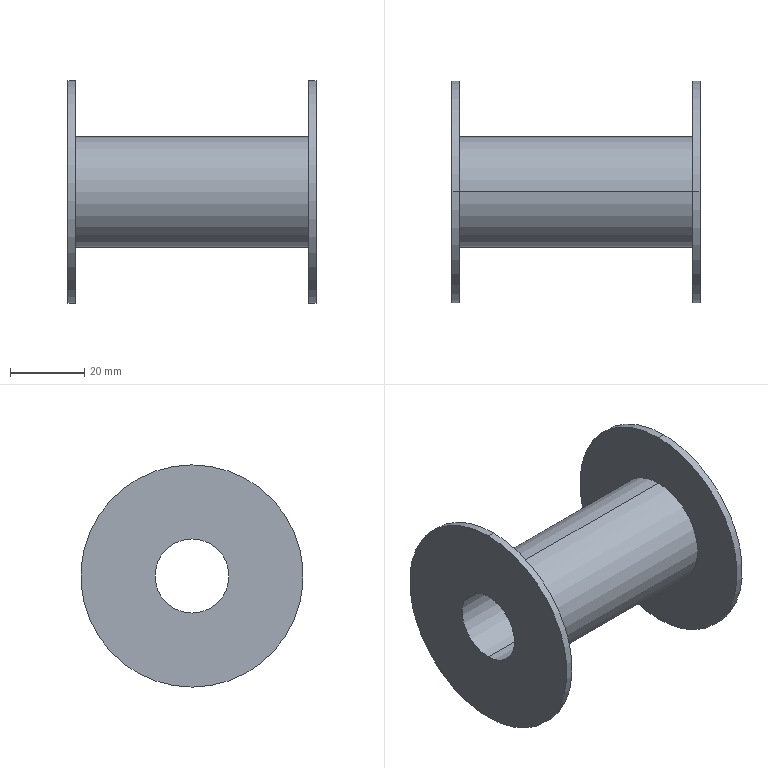Component | SolidWorks | AS-011-JG0101-2 | 1 solid | 12 faces | box 67 x 60 x 60 mm | volume 34793 mm3 | cylinder 8 | plane 4 | commonest cylinder face diameters 60 x4 30 x2 20 x2
build123d program:
from build123d import *


with BuildPart() as part:
    # Sketch1 → Revolve1 (revolve)
    with BuildSketch(Plane.XY, mode=Mode.PRIVATE) as revolve1_sk:
        Polygon((0, 10), (0, 30), (2, 30), (2, 15), (65, 15), (65, 30), (67, 30), (67, 10), align=None)
    revolve(revolve1_sk.sketch.rotate(Axis((0, 0, 0), (1, 0, 0)), 90), axis=Axis((0, 0, 0), (1, 0, 0)))


solid = part.part

# Placed as in the assembly
solid = solid.moved(Location((-51.5, -28, -112), (0, 0, 0)))
STEP:
#1=COLOUR_RGB('',0.7922,0.8196,0.9333);
#2=FILL_AREA_STYLE_COLOUR('',#1);
#3=FILL_AREA_STYLE('',(#2));
#4=SURFACE_STYLE_FILL_AREA(#3);
#5=SURFACE_SIDE_STYLE('',(#4));
#6=SURFACE_STYLE_USAGE(.BOTH.,#5);
#7=PRESENTATION_STYLE_ASSIGNMENT((#6));
#8=CARTESIAN_POINT('',(0.6102,-1.102,-3.228));
#9=VERTEX_POINT('',#8);
#10=CARTESIAN_POINT('',(0.6102,-1.103,-5.591));
#11=VERTEX_POINT('',#10);
#12=CARTESIAN_POINT('',(0.6102,-1.102,-4.409));
#13=DIRECTION('',(-1.,0.,0.));
#14=DIRECTION('',(0.,0.000194,1.));
#15=AXIS2_PLACEMENT_3D('',#12,#13,#14);
#16=CIRCLE('',#15,1.181);
#17=EDGE_CURVE('',#9,#11,#16,.T.);
#18=ORIENTED_EDGE('',*,*,#17,.T.);
#19=CARTESIAN_POINT('',(0.5315,-1.103,-5.591));
#20=VERTEX_POINT('',#19);
#21=CARTESIAN_POINT('',(-2.028,-1.103,-5.591));
#22=DIRECTION('',(-1.,0.,0.));
#23=VECTOR('',#22,39.37);
#24=LINE('',#21,#23);
#25=EDGE_CURVE('',#11,#20,#24,.T.);
#26=ORIENTED_EDGE('',*,*,#25,.T.);
#27=CARTESIAN_POINT('',(0.5315,-1.102,-3.228));
#28=VERTEX_POINT('',#27);
#29=CARTESIAN_POINT('',(0.5315,-1.102,-4.409));
#30=DIRECTION('',(-1.,0.,0.));
#31=DIRECTION('',(0.,0.000194,1.));
#32=AXIS2_PLACEMENT_3D('',#29,#30,#31);
#33=CIRCLE('',#32,1.181);
#34=EDGE_CURVE('',#28,#20,#33,.T.);
#35=ORIENTED_EDGE('',*,*,#34,.F.);
#36=CARTESIAN_POINT('',(-2.028,-1.102,-3.228));
#37=DIRECTION('',(-1.,0.,0.));
#38=VECTOR('',#37,39.37);
#39=LINE('',#36,#38);
#40=EDGE_CURVE('',#9,#28,#39,.T.);
#41=ORIENTED_EDGE('',*,*,#40,.F.);
#42=EDGE_LOOP('',(#18,#26,#35,#41));
#43=FACE_OUTER_BOUND('',#42,.T.);
#44=CARTESIAN_POINT('',(-2.028,-1.102,-4.409));
#45=DIRECTION('',(-1.,0.,0.));
#46=DIRECTION('',(0.,0.000194,1.));
#47=AXIS2_PLACEMENT_3D('',#44,#45,#46);
#48=CYLINDRICAL_SURFACE('',#47,1.181);
#49=ADVANCED_FACE('',(#43),#48,.T.);
#50=CARTESIAN_POINT('',(0.5315,-1.102,-3.819));
#51=VERTEX_POINT('',#50);
#52=CARTESIAN_POINT('',(0.5315,-1.102,-5.));
#53=VERTEX_POINT('',#52);
#54=CARTESIAN_POINT('',(0.5315,-1.102,-4.409));
#55=DIRECTION('',(-1.,0.,0.));
#56=DIRECTION('',(0.,0.000194,1.));
#57=AXIS2_PLACEMENT_3D('',#54,#55,#56);
#58=CIRCLE('',#57,0.5906);
#59=EDGE_CURVE('',#51,#53,#58,.T.);
#60=ORIENTED_EDGE('',*,*,#59,.T.);
#61=CARTESIAN_POINT('',(-1.949,-1.102,-5.));
#62=VERTEX_POINT('',#61);
#63=CARTESIAN_POINT('',(-2.028,-1.102,-5.));
#64=DIRECTION('',(-1.,0.,0.));
#65=VECTOR('',#64,39.37);
#66=LINE('',#63,#65);
#67=EDGE_CURVE('',#53,#62,#66,.T.);
#68=ORIENTED_EDGE('',*,*,#67,.T.);
#69=CARTESIAN_POINT('',(-1.949,-1.102,-3.819));
#70=VERTEX_POINT('',#69);
#71=CARTESIAN_POINT('',(-1.949,-1.102,-4.409));
#72=DIRECTION('',(-1.,0.,0.));
#73=DIRECTION('',(0.,0.000194,1.));
#74=AXIS2_PLACEMENT_3D('',#71,#72,#73);
#75=CIRCLE('',#74,0.5906);
#76=EDGE_CURVE('',#70,#62,#75,.T.);
#77=ORIENTED_EDGE('',*,*,#76,.F.);
#78=CARTESIAN_POINT('',(-2.028,-1.102,-3.819));
#79=DIRECTION('',(-1.,0.,0.));
#80=VECTOR('',#79,39.37);
#81=LINE('',#78,#80);
#82=EDGE_CURVE('',#51,#70,#81,.T.);
#83=ORIENTED_EDGE('',*,*,#82,.F.);
#84=EDGE_LOOP('',(#60,#68,#77,#83));
#85=FACE_OUTER_BOUND('',#84,.T.);
#86=CARTESIAN_POINT('',(-2.028,-1.102,-4.409));
#87=DIRECTION('',(-1.,0.,0.));
#88=DIRECTION('',(0.,0.000194,1.));
#89=AXIS2_PLACEMENT_3D('',#86,#87,#88);
#90=CYLINDRICAL_SURFACE('',#89,0.5906);
#91=ADVANCED_FACE('',(#85),#90,.T.);
#92=CARTESIAN_POINT('',(-1.949,-1.102,-3.228));
#93=VERTEX_POINT('',#92);
#94=CARTESIAN_POINT('',(-1.949,-1.103,-5.591));
#95=VERTEX_POINT('',#94);
#96=CARTESIAN_POINT('',(-1.949,-1.102,-4.409));
#97=DIRECTION('',(-1.,0.,0.));
#98=DIRECTION('',(0.,0.000194,1.));
#99=AXIS2_PLACEMENT_3D('',#96,#97,#98);
#100=CIRCLE('',#99,1.181);
#101=EDGE_CURVE('',#93,#95,#100,.T.);
#102=ORIENTED_EDGE('',*,*,#101,.T.);
#103=CARTESIAN_POINT('',(-2.028,-1.103,-5.591));
#104=VERTEX_POINT('',#103);
#105=CARTESIAN_POINT('',(-2.028,-1.103,-5.591));
#106=DIRECTION('',(-1.,0.,0.));
#107=VECTOR('',#106,39.37);
#108=LINE('',#105,#107);
#109=EDGE_CURVE('',#95,#104,#108,.T.);
#110=ORIENTED_EDGE('',*,*,#109,.T.);
#111=CARTESIAN_POINT('',(-2.028,-1.102,-3.228));
#112=VERTEX_POINT('',#111);
#113=CARTESIAN_POINT('',(-2.028,-1.102,-4.409));
#114=DIRECTION('',(-1.,0.,0.));
#115=DIRECTION('',(0.,0.000194,1.));
#116=AXIS2_PLACEMENT_3D('',#113,#114,#115);
#117=CIRCLE('',#116,1.181);
#118=EDGE_CURVE('',#112,#104,#117,.T.);
#119=ORIENTED_EDGE('',*,*,#118,.F.);
#120=CARTESIAN_POINT('',(-2.028,-1.102,-3.228));
#121=DIRECTION('',(-1.,0.,0.));
#122=VECTOR('',#121,39.37);
#123=LINE('',#120,#122);
#124=EDGE_CURVE('',#93,#112,#123,.T.);
#125=ORIENTED_EDGE('',*,*,#124,.F.);
#126=EDGE_LOOP('',(#102,#110,#119,#125));
#127=FACE_OUTER_BOUND('',#126,.T.);
#128=CARTESIAN_POINT('',(-2.028,-1.102,-4.409));
#129=DIRECTION('',(-1.,0.,0.));
#130=DIRECTION('',(0.,0.000194,1.));
#131=AXIS2_PLACEMENT_3D('',#128,#129,#130);
#132=CYLINDRICAL_SURFACE('',#131,1.181);
#133=ADVANCED_FACE('',(#127),#132,.T.);
#134=CARTESIAN_POINT('',(0.6102,-1.102,-4.803));
#135=VERTEX_POINT('',#134);
#136=CARTESIAN_POINT('',(0.6102,-1.102,-4.016));
#137=VERTEX_POINT('',#136);
#138=CARTESIAN_POINT('',(0.6102,-1.102,-4.409));
#139=DIRECTION('',(-1.,0.,0.));
#140=DIRECTION('',(0.,0.000194,1.));
#141=AXIS2_PLACEMENT_3D('',#138,#139,#140);
#142=CIRCLE('',#141,0.3937);
#143=EDGE_CURVE('',#135,#137,#142,.T.);
#144=ORIENTED_EDGE('',*,*,#143,.F.);
#145=CARTESIAN_POINT('',(-2.028,-1.102,-4.803));
#146=VERTEX_POINT('',#145);
#147=CARTESIAN_POINT('',(-2.028,-1.102,-4.803));
#148=DIRECTION('',(-1.,0.,0.));
#149=VECTOR('',#148,39.37);
#150=LINE('',#147,#149);
#151=EDGE_CURVE('',#135,#146,#150,.T.);
#152=ORIENTED_EDGE('',*,*,#151,.T.);
#153=CARTESIAN_POINT('',(-2.028,-1.102,-4.016));
#154=VERTEX_POINT('',#153);
#155=CARTESIAN_POINT('',(-2.028,-1.102,-4.409));
#156=DIRECTION('',(-1.,0.,0.));
#157=DIRECTION('',(0.,0.000194,1.));
#158=AXIS2_PLACEMENT_3D('',#155,#156,#157);
#159=CIRCLE('',#158,0.3937);
#160=EDGE_CURVE('',#146,#154,#159,.T.);
#161=ORIENTED_EDGE('',*,*,#160,.T.);
#162=CARTESIAN_POINT('',(-2.028,-1.102,-4.016));
#163=DIRECTION('',(-1.,0.,0.));
#164=VECTOR('',#163,39.37);
#165=LINE('',#162,#164);
#166=EDGE_CURVE('',#137,#154,#165,.T.);
#167=ORIENTED_EDGE('',*,*,#166,.F.);
#168=EDGE_LOOP('',(#144,#152,#161,#167));
#169=FACE_OUTER_BOUND('',#168,.T.);
#170=CARTESIAN_POINT('',(-2.028,-1.102,-4.409));
#171=DIRECTION('',(-1.,0.,0.));
#172=DIRECTION('',(0.,0.000194,1.));
#173=AXIS2_PLACEMENT_3D('',#170,#171,#172);
#174=CYLINDRICAL_SURFACE('',#173,0.3937);
#175=ADVANCED_FACE('',(#169),#174,.F.);
#176=ORIENTED_EDGE('',*,*,#151,.F.);
#177=CARTESIAN_POINT('',(0.6102,-1.102,-4.409));
#178=DIRECTION('',(-1.,0.,0.));
#179=DIRECTION('',(0.,0.000194,1.));
#180=AXIS2_PLACEMENT_3D('',#177,#178,#179);
#181=CIRCLE('',#180,0.3937);
#182=EDGE_CURVE('',#137,#135,#181,.T.);
#183=ORIENTED_EDGE('',*,*,#182,.F.);
#184=ORIENTED_EDGE('',*,*,#166,.T.);
#185=CARTESIAN_POINT('',(-2.028,-1.102,-4.409));
#186=DIRECTION('',(-1.,0.,0.));
#187=DIRECTION('',(0.,0.000194,1.));
#188=AXIS2_PLACEMENT_3D('',#185,#186,#187);
#189=CIRCLE('',#188,0.3937);
#190=EDGE_CURVE('',#154,#146,#189,.T.);
#191=ORIENTED_EDGE('',*,*,#190,.T.);
#192=EDGE_LOOP('',(#176,#183,#184,#191));
#193=FACE_OUTER_BOUND('',#192,.T.);
#194=CARTESIAN_POINT('',(-2.028,-1.102,-4.409));
#195=DIRECTION('',(-1.,0.,0.));
#196=DIRECTION('',(0.,0.000194,1.));
#197=AXIS2_PLACEMENT_3D('',#194,#195,#196);
#198=CYLINDRICAL_SURFACE('',#197,0.3937);
#199=ADVANCED_FACE('',(#193),#198,.F.);
#200=ORIENTED_EDGE('',*,*,#190,.F.);
#201=ORIENTED_EDGE('',*,*,#160,.F.);
#202=EDGE_LOOP('',(#200,#201));
#203=FACE_BOUND('',#202,.T.);
#204=ORIENTED_EDGE('',*,*,#118,.T.);
#205=CARTESIAN_POINT('',(-2.028,-1.102,-4.409));
#206=DIRECTION('',(-1.,0.,0.));
#207=DIRECTION('',(0.,0.000194,1.));
#208=AXIS2_PLACEMENT_3D('',#205,#206,#207);
#209=CIRCLE('',#208,1.181);
#210=EDGE_CURVE('',#104,#112,#209,.T.);
#211=ORIENTED_EDGE('',*,*,#210,.T.);
#212=EDGE_LOOP('',(#204,#211));
#213=FACE_OUTER_BOUND('',#212,.T.);
#214=CARTESIAN_POINT('',(-2.028,-0.7087,-4.41));
#215=DIRECTION('',(1.,-0.,-0.));
#216=DIRECTION('',(-0.,-0.000194,-1.));
#217=AXIS2_PLACEMENT_3D('',#214,#215,#216);
#218=PLANE('',#217);
#219=ADVANCED_FACE('',(#203,#213),#218,.F.);
#220=ORIENTED_EDGE('',*,*,#109,.F.);
#221=CARTESIAN_POINT('',(-1.949,-1.102,-4.409));
#222=DIRECTION('',(-1.,0.,0.));
#223=DIRECTION('',(0.,0.000194,1.));
#224=AXIS2_PLACEMENT_3D('',#221,#222,#223);
#225=CIRCLE('',#224,1.181);
#226=EDGE_CURVE('',#95,#93,#225,.T.);
#227=ORIENTED_EDGE('',*,*,#226,.T.);
#228=ORIENTED_EDGE('',*,*,#124,.T.);
#229=ORIENTED_EDGE('',*,*,#210,.F.);
#230=EDGE_LOOP('',(#220,#227,#228,#229));
#231=FACE_OUTER_BOUND('',#230,.T.);
#232=CARTESIAN_POINT('',(-2.028,-1.102,-4.409));
#233=DIRECTION('',(-1.,0.,0.));
#234=DIRECTION('',(0.,0.000194,1.));
#235=AXIS2_PLACEMENT_3D('',#232,#233,#234);
#236=CYLINDRICAL_SURFACE('',#235,1.181);
#237=ADVANCED_FACE('',(#231),#236,.T.);
#238=ORIENTED_EDGE('',*,*,#101,.F.);
#239=ORIENTED_EDGE('',*,*,#226,.F.);
#240=EDGE_LOOP('',(#238,#239));
#241=FACE_OUTER_BOUND('',#240,.T.);
#242=ORIENTED_EDGE('',*,*,#76,.T.);
#243=CARTESIAN_POINT('',(-1.949,-1.102,-4.409));
#244=DIRECTION('',(-1.,0.,0.));
#245=DIRECTION('',(0.,0.000194,1.));
#246=AXIS2_PLACEMENT_3D('',#243,#244,#245);
#247=CIRCLE('',#246,0.5906);
#248=EDGE_CURVE('',#62,#70,#247,.T.);
#249=ORIENTED_EDGE('',*,*,#248,.T.);
#250=EDGE_LOOP('',(#242,#249));
#251=FACE_BOUND('',#250,.T.);
#252=CARTESIAN_POINT('',(-1.949,-0.5118,-4.41));
#253=DIRECTION('',(-1.,0.,0.));
#254=DIRECTION('',(0.,0.000194,1.));
#255=AXIS2_PLACEMENT_3D('',#252,#253,#254);
#256=PLANE('',#255);
#257=ADVANCED_FACE('',(#241,#251),#256,.F.);
#258=ORIENTED_EDGE('',*,*,#67,.F.);
#259=CARTESIAN_POINT('',(0.5315,-1.102,-4.409));
#260=DIRECTION('',(-1.,0.,0.));
#261=DIRECTION('',(0.,0.000194,1.));
#262=AXIS2_PLACEMENT_3D('',#259,#260,#261);
#263=CIRCLE('',#262,0.5906);
#264=EDGE_CURVE('',#53,#51,#263,.T.);
#265=ORIENTED_EDGE('',*,*,#264,.T.);
#266=ORIENTED_EDGE('',*,*,#82,.T.);
#267=ORIENTED_EDGE('',*,*,#248,.F.);
#268=EDGE_LOOP('',(#258,#265,#266,#267));
#269=FACE_OUTER_BOUND('',#268,.T.);
#270=CARTESIAN_POINT('',(-2.028,-1.102,-4.409));
#271=DIRECTION('',(-1.,0.,0.));
#272=DIRECTION('',(0.,0.000194,1.));
#273=AXIS2_PLACEMENT_3D('',#270,#271,#272);
#274=CYLINDRICAL_SURFACE('',#273,0.5906);
#275=ADVANCED_FACE('',(#269),#274,.T.);
#276=ORIENTED_EDGE('',*,*,#59,.F.);
#277=ORIENTED_EDGE('',*,*,#264,.F.);
#278=EDGE_LOOP('',(#276,#277));
#279=FACE_BOUND('',#278,.T.);
#280=ORIENTED_EDGE('',*,*,#34,.T.);
#281=CARTESIAN_POINT('',(0.5315,-1.102,-4.409));
#282=DIRECTION('',(-1.,0.,0.));
#283=DIRECTION('',(0.,0.000194,1.));
#284=AXIS2_PLACEMENT_3D('',#281,#282,#283);
#285=CIRCLE('',#284,1.181);
#286=EDGE_CURVE('',#20,#28,#285,.T.);
#287=ORIENTED_EDGE('',*,*,#286,.T.);
#288=EDGE_LOOP('',(#280,#287));
#289=FACE_OUTER_BOUND('',#288,.T.);
#290=CARTESIAN_POINT('',(0.5315,-0.5118,-4.41));
#291=DIRECTION('',(1.,-0.,-0.));
#292=DIRECTION('',(-0.,-0.000194,-1.));
#293=AXIS2_PLACEMENT_3D('',#290,#291,#292);
#294=PLANE('',#293);
#295=ADVANCED_FACE('',(#279,#289),#294,.F.);
#296=ORIENTED_EDGE('',*,*,#25,.F.);
#297=CARTESIAN_POINT('',(0.6102,-1.102,-4.409));
#298=DIRECTION('',(-1.,0.,0.));
#299=DIRECTION('',(0.,0.000194,1.));
#300=AXIS2_PLACEMENT_3D('',#297,#298,#299);
#301=CIRCLE('',#300,1.181);
#302=EDGE_CURVE('',#11,#9,#301,.T.);
#303=ORIENTED_EDGE('',*,*,#302,.T.);
#304=ORIENTED_EDGE('',*,*,#40,.T.);
#305=ORIENTED_EDGE('',*,*,#286,.F.);
#306=EDGE_LOOP('',(#296,#303,#304,#305));
#307=FACE_OUTER_BOUND('',#306,.T.);
#308=CARTESIAN_POINT('',(-2.028,-1.102,-4.409));
#309=DIRECTION('',(-1.,0.,0.));
#310=DIRECTION('',(0.,0.000194,1.));
#311=AXIS2_PLACEMENT_3D('',#308,#309,#310);
#312=CYLINDRICAL_SURFACE('',#311,1.181);
#313=ADVANCED_FACE('',(#307),#312,.T.);
#314=ORIENTED_EDGE('',*,*,#17,.F.);
#315=ORIENTED_EDGE('',*,*,#302,.F.);
#316=EDGE_LOOP('',(#314,#315));
#317=FACE_OUTER_BOUND('',#316,.T.);
#318=ORIENTED_EDGE('',*,*,#182,.T.);
#319=ORIENTED_EDGE('',*,*,#143,.T.);
#320=EDGE_LOOP('',(#318,#319));
#321=FACE_BOUND('',#320,.T.);
#322=CARTESIAN_POINT('',(0.6102,-0.7087,-4.41));
#323=DIRECTION('',(-1.,0.,0.));
#324=DIRECTION('',(0.,0.000194,1.));
#325=AXIS2_PLACEMENT_3D('',#322,#323,#324);
#326=PLANE('',#325);
#327=ADVANCED_FACE('',(#317,#321),#326,.F.);
#328=CLOSED_SHELL('',(#49,#91,#133,#175,#199,#219,#237,#257,#275,#295,#313,#327));
#329=MANIFOLD_SOLID_BREP('',#328);
#330=STYLED_ITEM('',(#7),#329);
#331=(LENGTH_UNIT()NAMED_UNIT(*)SI_UNIT($,.METRE.));
#332=LENGTH_MEASURE_WITH_UNIT(LENGTH_MEASURE(0.0254),#331);
#333=DIMENSIONAL_EXPONENTS(1.,0.,0.,0.,0.,0.,0.);
#334=(CONVERSION_BASED_UNIT('',#332)LENGTH_UNIT()NAMED_UNIT(#333));
#335=UNCERTAINTY_MEASURE_WITH_UNIT(LENGTH_MEASURE(0.00001),#334,'','');
#336=(NAMED_UNIT(*)PLANE_ANGLE_UNIT()SI_UNIT($,.RADIAN.));
#337=(NAMED_UNIT(*)SI_UNIT($,.STERADIAN.)SOLID_ANGLE_UNIT());
#338=(GEOMETRIC_REPRESENTATION_CONTEXT(3)GLOBAL_UNCERTAINTY_ASSIGNED_CONTEXT((#335))GLOBAL_UNIT_ASSIGNED_CONTEXT((#334,#336,#337))REPRESENTATION_CONTEXT('',''));
#339=MECHANICAL_DESIGN_GEOMETRIC_PRESENTATION_REPRESENTATION('',(#330),#338);
#340=CARTESIAN_POINT('',(0.,0.,0.));
#341=DIRECTION('',(0.,0.,1.));
#342=DIRECTION('',(1.,0.,0.));
#343=AXIS2_PLACEMENT_3D('',#340,#341,#342);
#344=(LENGTH_UNIT()NAMED_UNIT(*)SI_UNIT($,.METRE.));
#345=LENGTH_MEASURE_WITH_UNIT(LENGTH_MEASURE(0.0254),#344);
#346=DIMENSIONAL_EXPONENTS(1.,0.,0.,0.,0.,0.,0.);
#347=(CONVERSION_BASED_UNIT('',#345)LENGTH_UNIT()NAMED_UNIT(#346));
#348=UNCERTAINTY_MEASURE_WITH_UNIT(LENGTH_MEASURE(0.00001),#347,'','');
#349=(NAMED_UNIT(*)PLANE_ANGLE_UNIT()SI_UNIT($,.RADIAN.));
#350=(NAMED_UNIT(*)SI_UNIT($,.STERADIAN.)SOLID_ANGLE_UNIT());
#351=(GEOMETRIC_REPRESENTATION_CONTEXT(3)GLOBAL_UNCERTAINTY_ASSIGNED_CONTEXT((#348))GLOBAL_UNIT_ASSIGNED_CONTEXT((#347,#349,#350))REPRESENTATION_CONTEXT('',''));
#352=ADVANCED_BREP_SHAPE_REPRESENTATION('',(#329,#343),#351);
#353=PRESENTATION_LAYER_ASSIGNMENT('','',(#330));